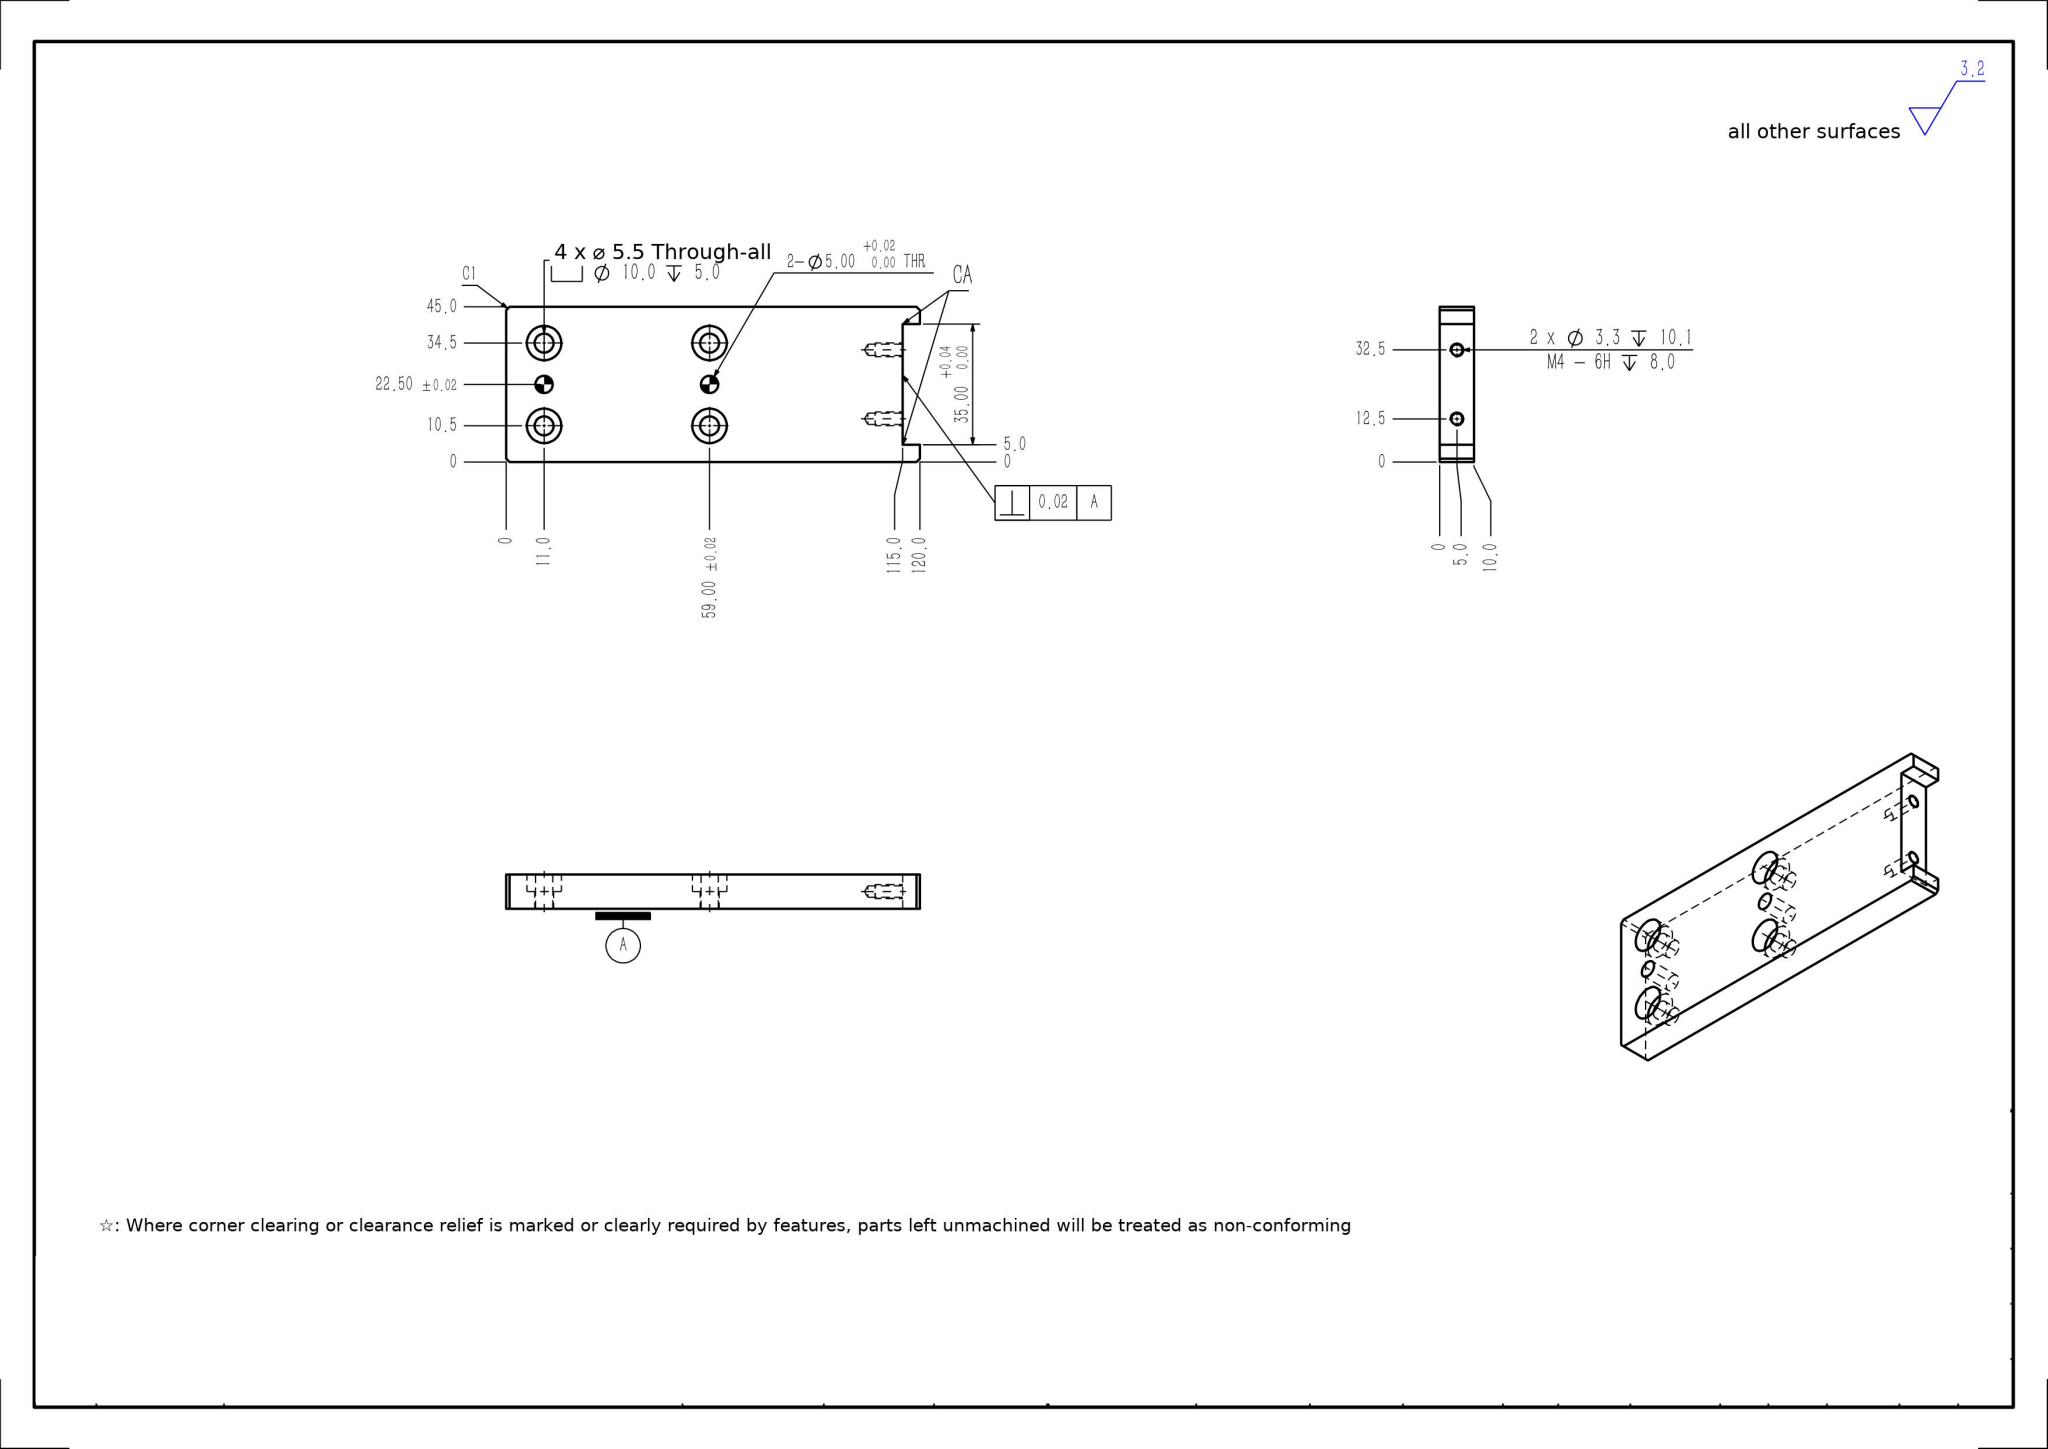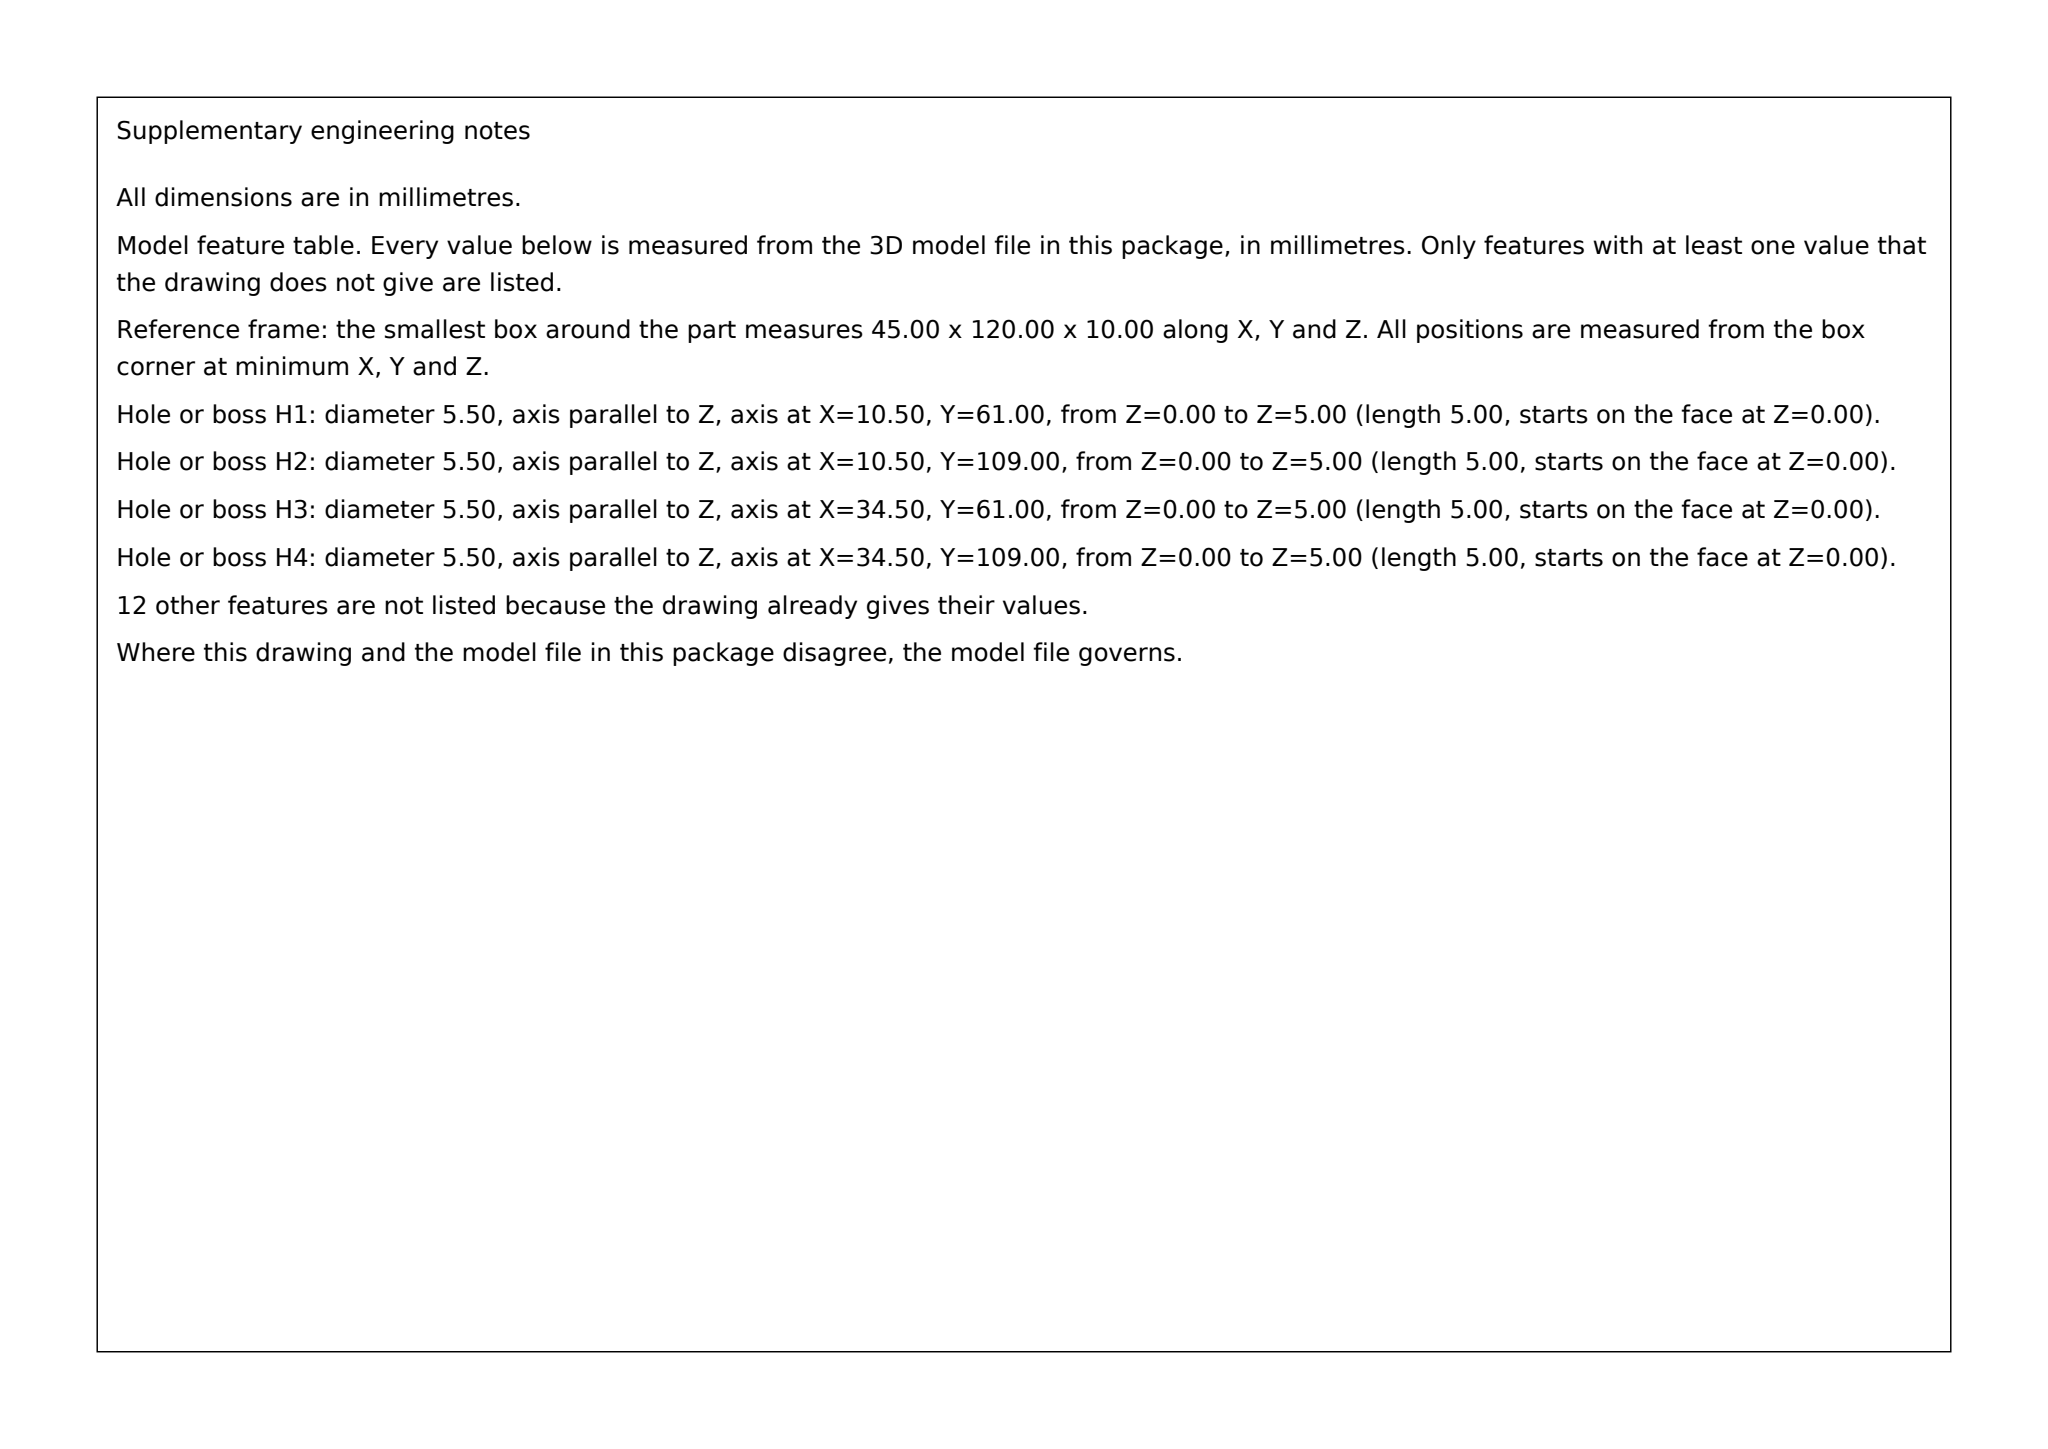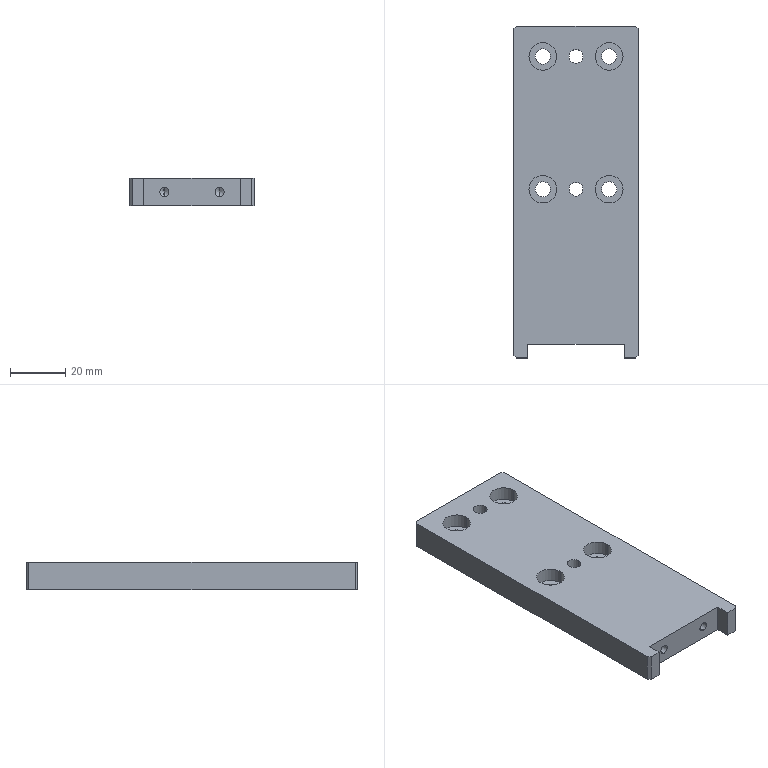Part | SolidWorks | mm | 1 solid | 46 faces | box 45 x 120 x 10 mm | volume 49613 mm3 | cylinder 24 | plane 18 | cone 4 | commonest cylinder face diameters 10 x8 5.5 x8 3.3 x4 5 x4
build123d program:
from build123d import *

# Parameters (mm, degrees)
SKETCH1_W                                       = 10
SKETCH1_H                                       = 120
BOSS_EXTRUDE1_DEPTH                             = 22.5
SKETCH3_W                                       = 35
SKETCH3_H                                       = 5
CUT_EXTRUDE1_DEPTH                              = 65.856
CHAMFER1_SIZE                                   = 1
M5_HEX_SOCKET_HEAD_CAP_SCREW_CBORE1_D           = 5.5
M5_HEX_SOCKET_HEAD_CAP_SCREW_CBORE1_CBORE_D     = 10
M5_HEX_SOCKET_HEAD_CAP_SCREW_CBORE1_CBORE_DEPTH = 5
SIZE_MM_DOWEL_HOLE1_D                           = 5
M4_TAPPED_HOLE1_D                               = 3.3
M4_TAPPED_HOLE1_DEPTH                           = 10.1
M4_TAPPED_HOLE1_TIP                             = 0.9914


with BuildPart() as part:
    # Sketch1 → Boss-Extrude1 (new, symmetric)
    with BuildSketch(Plane(origin=(0, 0, 0), x_dir=(0, 0, -1), z_dir=(1, 0, 0))):
        Rectangle(SKETCH1_W, SKETCH1_H)
    extrude(amount=BOSS_EXTRUDE1_DEPTH, both=True)

    # Sketch3 → Cut-Extrude1 (cut, through all)
    with BuildSketch(Plane.XY.offset(5)):
        with Locations((0, -57.5)):
            Rectangle(SKETCH3_W, SKETCH3_H)
    extrude(amount=-CUT_EXTRUDE1_DEPTH, mode=Mode.SUBTRACT)

    # Chamfer1
    chamfer1_edges = [part.edges().sort_by_distance(p)[0] for p in [
        (22.5, -60, 0),
        (-22.5, -60, 0),
        (-22.5, 60, 0),
        (22.5, 60, 0),
    ]]
    chamfer(chamfer1_edges, length=CHAMFER1_SIZE)

    # M5 Hex Socket Head Cap Screw CBORE1 (through all)
    with Locations(Plane.XY.offset(5)):
        with Locations((12, 49), (-12, 49), (12, 1), (-12, 1)):
            CounterBoreHole(M5_HEX_SOCKET_HEAD_CAP_SCREW_CBORE1_D / 2, M5_HEX_SOCKET_HEAD_CAP_SCREW_CBORE1_CBORE_D / 2, M5_HEX_SOCKET_HEAD_CAP_SCREW_CBORE1_CBORE_DEPTH)

    # Size mm Dowel Hole1 (through all)
    with Locations(Plane.XY.offset(5)):
        with Locations((0, 49), (0, 1)):
            Hole(SIZE_MM_DOWEL_HOLE1_D / 2)

    # M4 Tapped Hole1
    with Locations(Plane(origin=(0, -55, 0), x_dir=(-1, 0, 0), z_dir=(0, -1, 0))):
        with Locations((10, 0), (-10, 0)):
            Hole(M4_TAPPED_HOLE1_D / 2, depth=M4_TAPPED_HOLE1_DEPTH)
            with Locations((0, 0, -(M4_TAPPED_HOLE1_DEPTH + M4_TAPPED_HOLE1_TIP / 2))):  # 118° drill point
                Cone(0, M4_TAPPED_HOLE1_D / 2, M4_TAPPED_HOLE1_TIP, mode=Mode.SUBTRACT)


solid = part.part